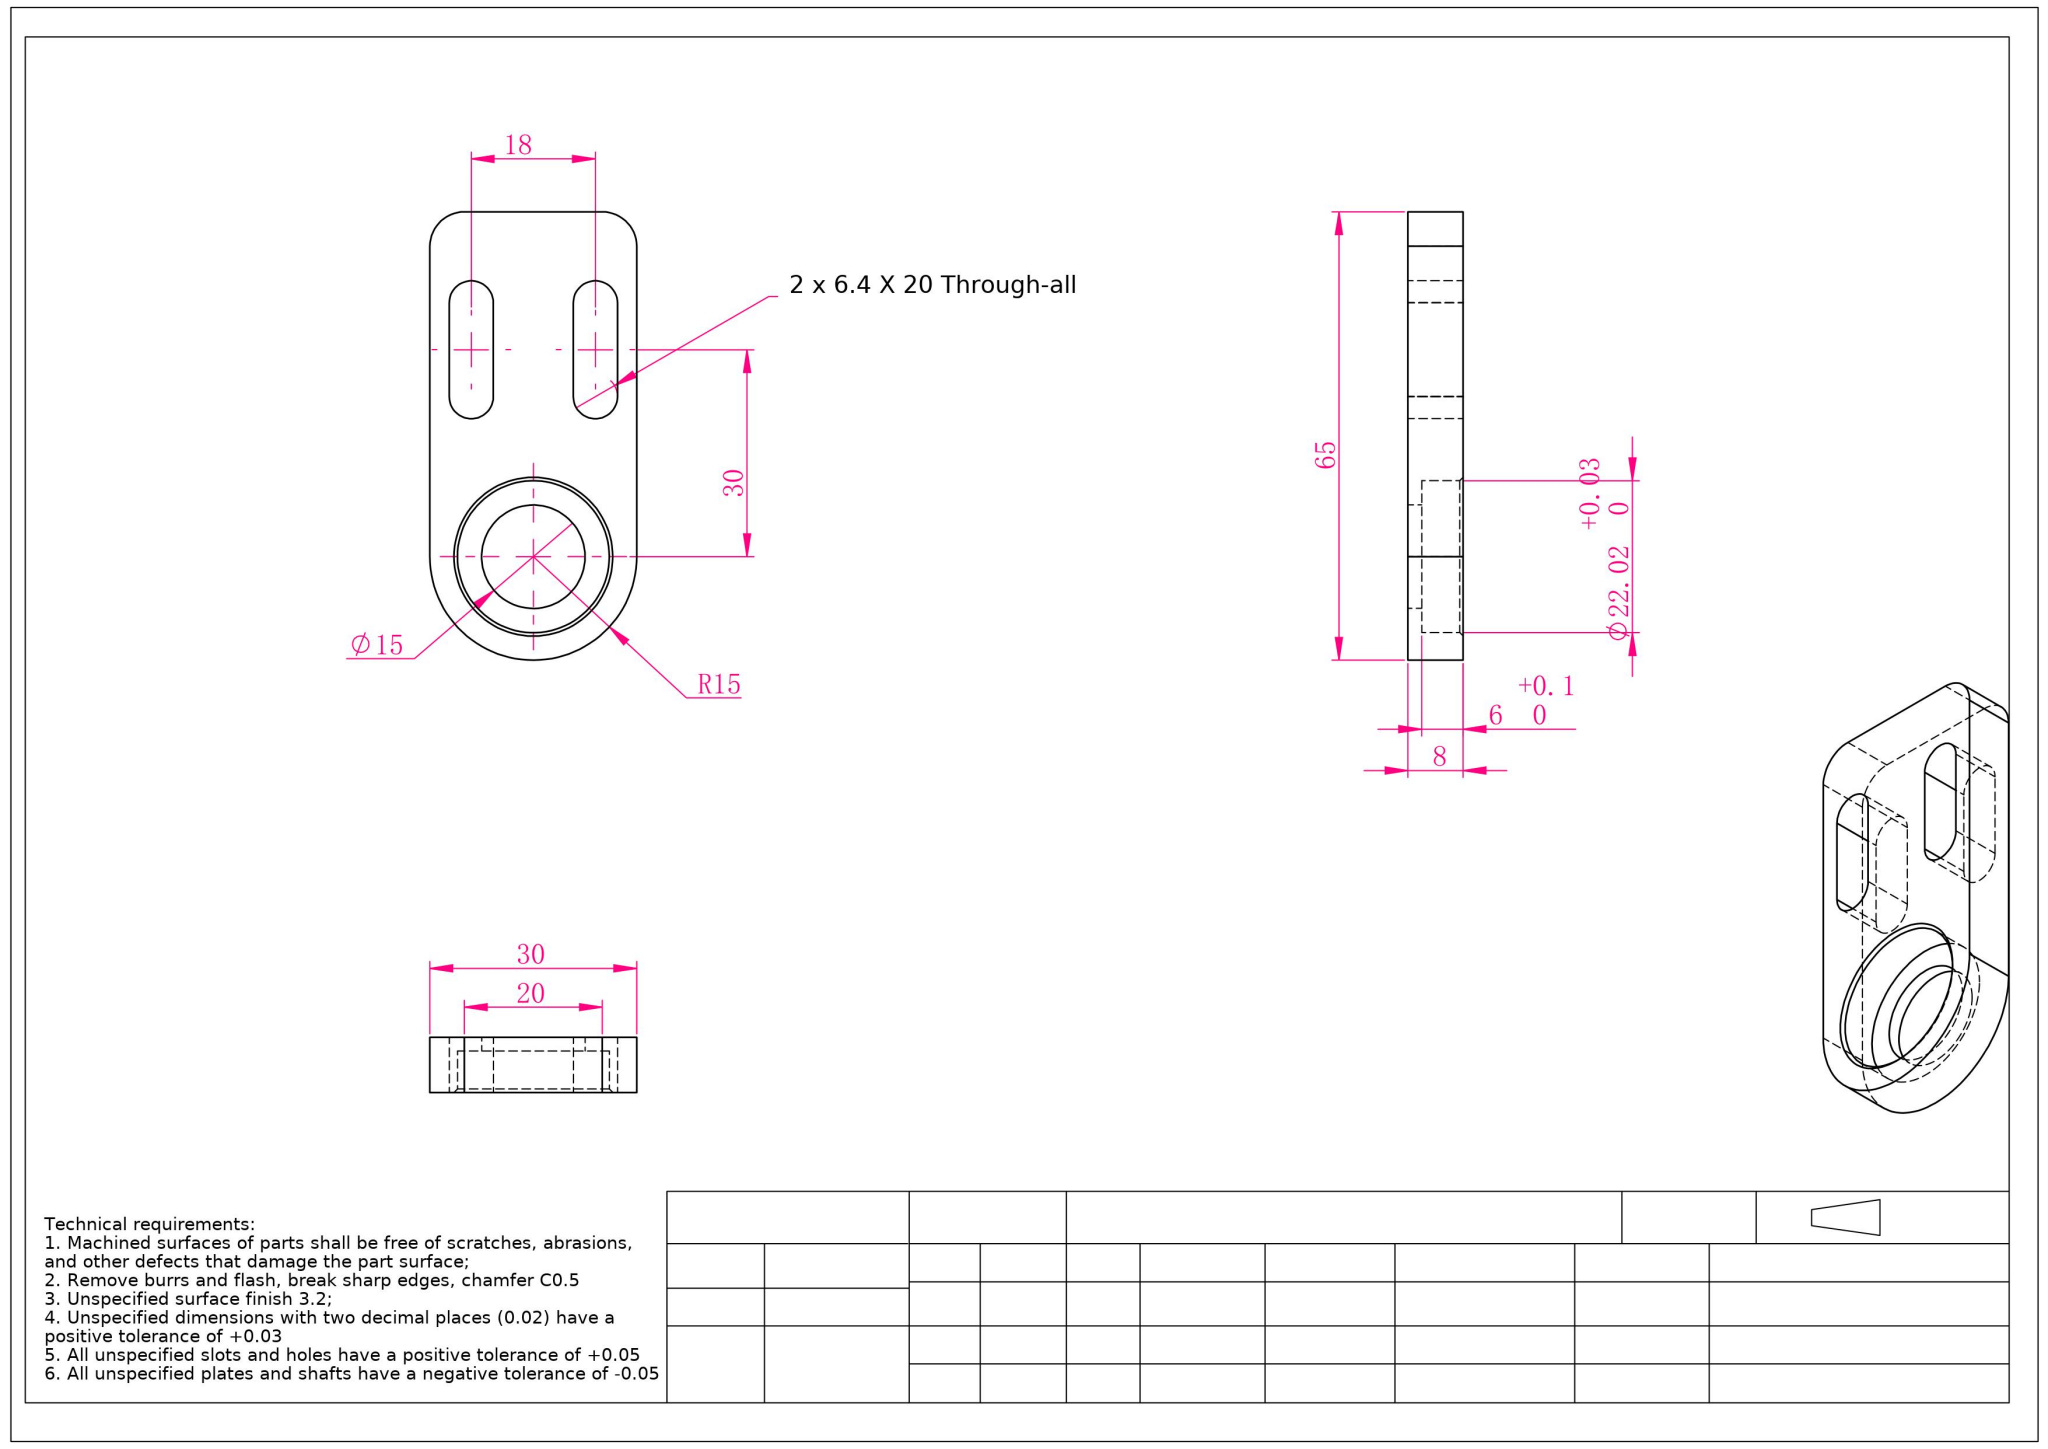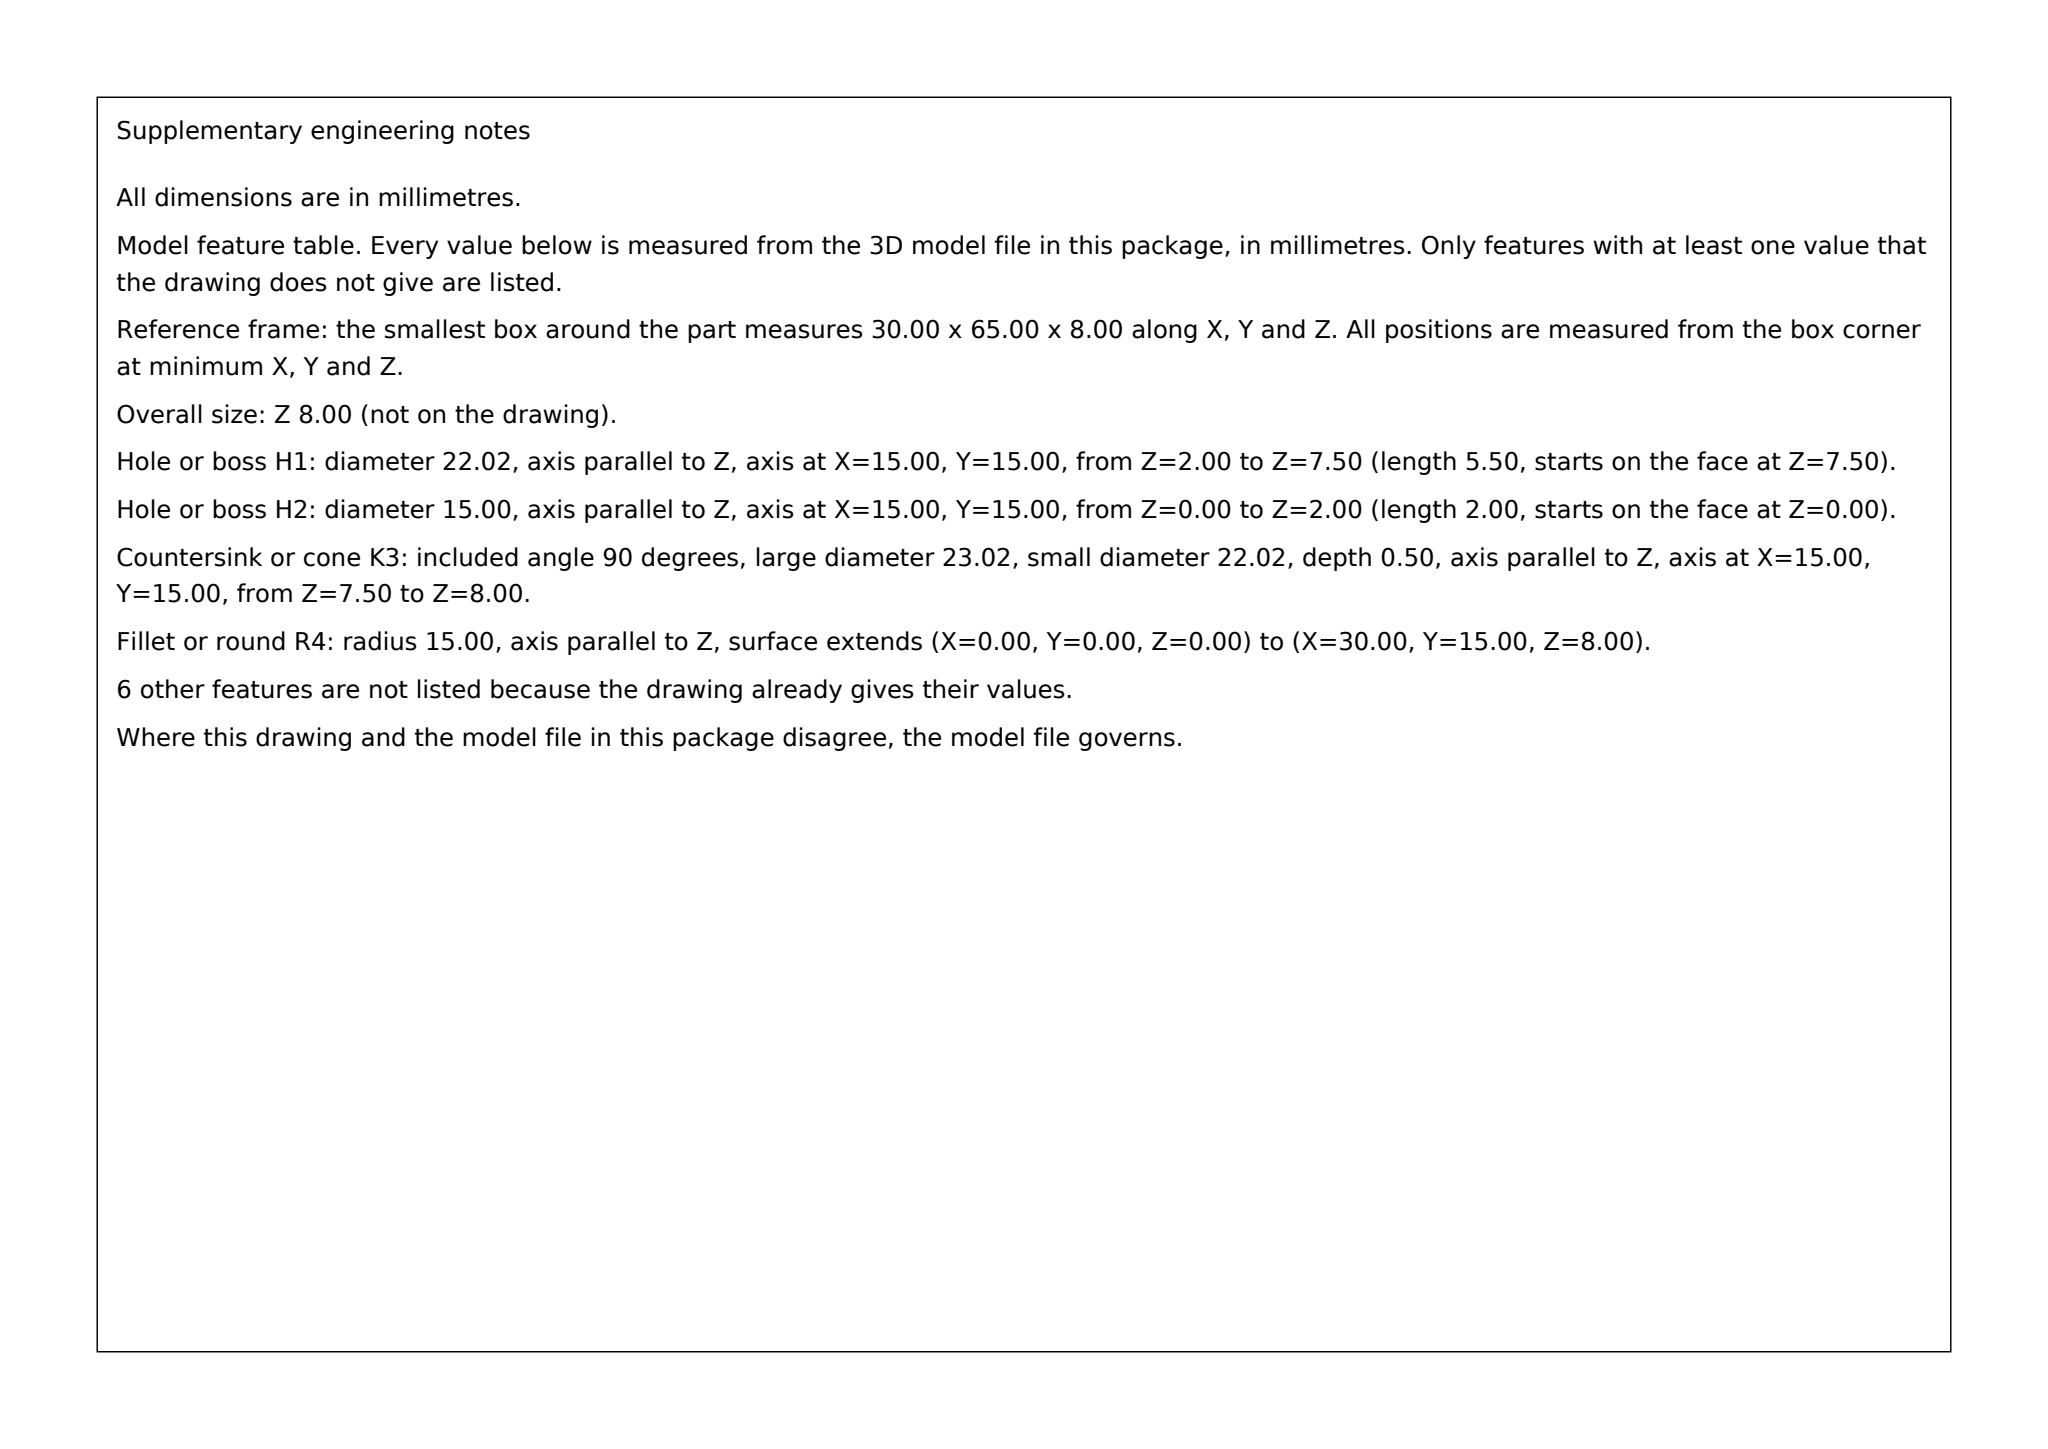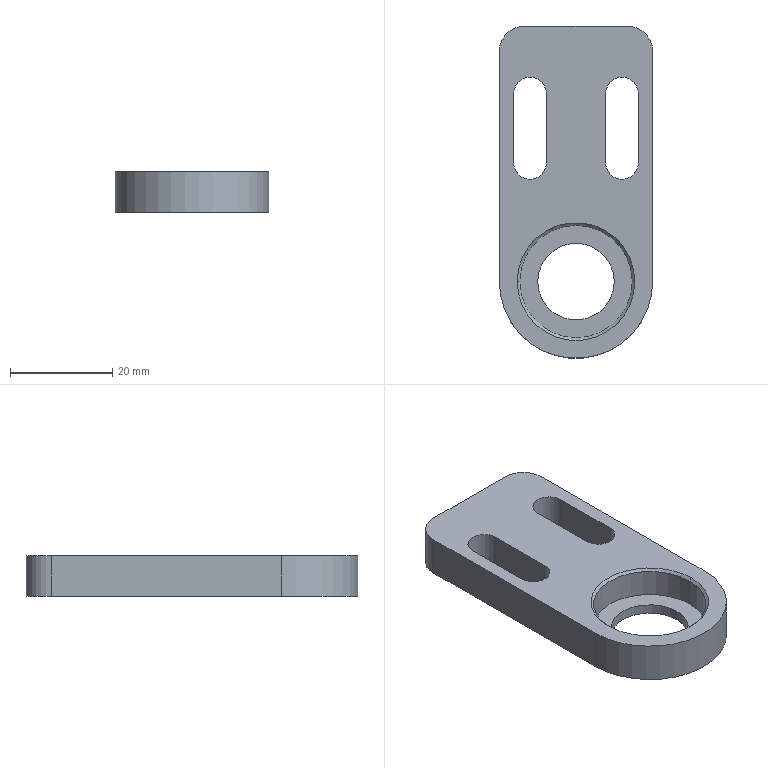Part | SolidWorks | mm | 1 solid | 23 faces | box 30 x 65 x 8 mm | volume 10187 mm3 | cylinder 11 | plane 10 | cone 2 | commonest cylinder face diameters 6.4 x4 22.02 x2 15 x2 10 x2 30 x1
STEP:
#1=CARTESIAN_POINT('',(-11.01,0.,3.5));
#2=VERTEX_POINT('',#1);
#3=CARTESIAN_POINT('',(11.01,0.,3.5));
#4=VERTEX_POINT('',#3);
#5=CARTESIAN_POINT('',(0.,0.,3.5));
#6=DIRECTION('',(0.,0.,1.));
#7=DIRECTION('',(1.,0.,0.));
#8=AXIS2_PLACEMENT_3D('',#5,#6,#7);
#9=CIRCLE('',#8,11.01);
#10=EDGE_CURVE('',#2,#4,#9,.T.);
#11=ORIENTED_EDGE('',*,*,#10,.F.);
#12=CARTESIAN_POINT('',(-11.51,0.,4.));
#13=VERTEX_POINT('',#12);
#14=CARTESIAN_POINT('',(-11.01,0.,3.5));
#15=DIRECTION('',(-0.7071,0.,0.7071));
#16=VECTOR('',#15,1000.);
#17=LINE('',#14,#16);
#18=EDGE_CURVE('',#2,#13,#17,.T.);
#19=ORIENTED_EDGE('',*,*,#18,.T.);
#20=CARTESIAN_POINT('',(11.51,0.,4.));
#21=VERTEX_POINT('',#20);
#22=CARTESIAN_POINT('',(0.,0.,4.));
#23=DIRECTION('',(0.,0.,-1.));
#24=DIRECTION('',(1.,0.,0.));
#25=AXIS2_PLACEMENT_3D('',#22,#23,#24);
#26=CIRCLE('',#25,11.51);
#27=EDGE_CURVE('',#21,#13,#26,.T.);
#28=ORIENTED_EDGE('',*,*,#27,.F.);
#29=CARTESIAN_POINT('',(11.01,0.,3.5));
#30=DIRECTION('',(0.7071,0.,0.7071));
#31=VECTOR('',#30,1000.);
#32=LINE('',#29,#31);
#33=EDGE_CURVE('',#4,#21,#32,.T.);
#34=ORIENTED_EDGE('',*,*,#33,.F.);
#35=EDGE_LOOP('',(#11,#19,#28,#34));
#36=FACE_OUTER_BOUND('',#35,.T.);
#37=CARTESIAN_POINT('',(0.,0.,3.5));
#38=DIRECTION('',(0.,0.,1.));
#39=DIRECTION('',(1.,0.,0.));
#40=AXIS2_PLACEMENT_3D('',#37,#38,#39);
#41=CONICAL_SURFACE('',#40,11.01,0.7854);
#42=ADVANCED_FACE('',(#36),#41,.F.);
#43=CARTESIAN_POINT('',(-11.01,0.,-2.));
#44=VERTEX_POINT('',#43);
#45=CARTESIAN_POINT('',(11.01,0.,-2.));
#46=VERTEX_POINT('',#45);
#47=CARTESIAN_POINT('',(0.,0.,-2.));
#48=DIRECTION('',(0.,0.,1.));
#49=DIRECTION('',(1.,0.,0.));
#50=AXIS2_PLACEMENT_3D('',#47,#48,#49);
#51=CIRCLE('',#50,11.01);
#52=EDGE_CURVE('',#44,#46,#51,.T.);
#53=ORIENTED_EDGE('',*,*,#52,.F.);
#54=CARTESIAN_POINT('',(-11.01,0.,-2.));
#55=DIRECTION('',(0.,0.,1.));
#56=VECTOR('',#55,1000.);
#57=LINE('',#54,#56);
#58=EDGE_CURVE('',#44,#2,#57,.T.);
#59=ORIENTED_EDGE('',*,*,#58,.T.);
#60=ORIENTED_EDGE('',*,*,#10,.T.);
#61=CARTESIAN_POINT('',(11.01,0.,-2.));
#62=DIRECTION('',(0.,0.,1.));
#63=VECTOR('',#62,1000.);
#64=LINE('',#61,#63);
#65=EDGE_CURVE('',#46,#4,#64,.T.);
#66=ORIENTED_EDGE('',*,*,#65,.F.);
#67=EDGE_LOOP('',(#53,#59,#60,#66));
#68=FACE_OUTER_BOUND('',#67,.T.);
#69=CARTESIAN_POINT('',(0.,0.,-2.));
#70=DIRECTION('',(0.,0.,1.));
#71=DIRECTION('',(1.,0.,0.));
#72=AXIS2_PLACEMENT_3D('',#69,#70,#71);
#73=CYLINDRICAL_SURFACE('',#72,11.01);
#74=ADVANCED_FACE('',(#68),#73,.F.);
#75=CARTESIAN_POINT('',(-7.5,0.,-2.));
#76=VERTEX_POINT('',#75);
#77=CARTESIAN_POINT('',(7.5,0.,-2.));
#78=VERTEX_POINT('',#77);
#79=CARTESIAN_POINT('',(0.,0.,-2.));
#80=DIRECTION('',(0.,0.,1.));
#81=DIRECTION('',(1.,0.,0.));
#82=AXIS2_PLACEMENT_3D('',#79,#80,#81);
#83=CIRCLE('',#82,7.5);
#84=EDGE_CURVE('',#76,#78,#83,.T.);
#85=ORIENTED_EDGE('',*,*,#84,.T.);
#86=CARTESIAN_POINT('',(7.5,0.,-4.));
#87=VERTEX_POINT('',#86);
#88=CARTESIAN_POINT('',(7.5,0.,4.));
#89=DIRECTION('',(0.,0.,-1.));
#90=VECTOR('',#89,1000.);
#91=LINE('',#88,#90);
#92=EDGE_CURVE('',#78,#87,#91,.T.);
#93=ORIENTED_EDGE('',*,*,#92,.T.);
#94=CARTESIAN_POINT('',(-7.5,0.,-4.));
#95=VERTEX_POINT('',#94);
#96=CARTESIAN_POINT('',(0.,0.,-4.));
#97=DIRECTION('',(0.,0.,1.));
#98=DIRECTION('',(1.,0.,0.));
#99=AXIS2_PLACEMENT_3D('',#96,#97,#98);
#100=CIRCLE('',#99,7.5);
#101=EDGE_CURVE('',#95,#87,#100,.T.);
#102=ORIENTED_EDGE('',*,*,#101,.F.);
#103=CARTESIAN_POINT('',(-7.5,0.,4.));
#104=DIRECTION('',(0.,0.,-1.));
#105=VECTOR('',#104,1000.);
#106=LINE('',#103,#105);
#107=EDGE_CURVE('',#76,#95,#106,.T.);
#108=ORIENTED_EDGE('',*,*,#107,.F.);
#109=EDGE_LOOP('',(#85,#93,#102,#108));
#110=FACE_OUTER_BOUND('',#109,.T.);
#111=CARTESIAN_POINT('',(0.,0.,4.));
#112=DIRECTION('',(0.,0.,-1.));
#113=DIRECTION('',(-1.,0.,0.));
#114=AXIS2_PLACEMENT_3D('',#111,#112,#113);
#115=CYLINDRICAL_SURFACE('',#114,7.5);
#116=ADVANCED_FACE('',(#110),#115,.F.);
#117=CARTESIAN_POINT('',(12.2,23.2,-4.));
#118=VERTEX_POINT('',#117);
#119=CARTESIAN_POINT('',(5.8,23.2,-4.));
#120=VERTEX_POINT('',#119);
#121=CARTESIAN_POINT('',(9.,23.2,-4.));
#122=DIRECTION('',(0.,0.,-1.));
#123=DIRECTION('',(-1.,0.,0.));
#124=AXIS2_PLACEMENT_3D('',#121,#122,#123);
#125=CIRCLE('',#124,3.2);
#126=EDGE_CURVE('',#118,#120,#125,.T.);
#127=ORIENTED_EDGE('',*,*,#126,.F.);
#128=CARTESIAN_POINT('',(12.2,36.8,-4.));
#129=VERTEX_POINT('',#128);
#130=CARTESIAN_POINT('',(12.2,23.2,-4.));
#131=DIRECTION('',(0.,1.,0.));
#132=VECTOR('',#131,1000.);
#133=LINE('',#130,#132);
#134=EDGE_CURVE('',#118,#129,#133,.T.);
#135=ORIENTED_EDGE('',*,*,#134,.T.);
#136=CARTESIAN_POINT('',(5.8,36.8,-4.));
#137=VERTEX_POINT('',#136);
#138=CARTESIAN_POINT('',(9.,36.8,-4.));
#139=DIRECTION('',(0.,0.,-1.));
#140=DIRECTION('',(-1.,0.,0.));
#141=AXIS2_PLACEMENT_3D('',#138,#139,#140);
#142=CIRCLE('',#141,3.2);
#143=EDGE_CURVE('',#137,#129,#142,.T.);
#144=ORIENTED_EDGE('',*,*,#143,.F.);
#145=CARTESIAN_POINT('',(5.8,23.2,-4.));
#146=DIRECTION('',(0.,1.,0.));
#147=VECTOR('',#146,1000.);
#148=LINE('',#145,#147);
#149=EDGE_CURVE('',#120,#137,#148,.T.);
#150=ORIENTED_EDGE('',*,*,#149,.F.);
#151=EDGE_LOOP('',(#127,#135,#144,#150));
#152=FACE_BOUND('',#151,.T.);
#153=ORIENTED_EDGE('',*,*,#101,.T.);
#154=CARTESIAN_POINT('',(0.,0.,-4.));
#155=DIRECTION('',(0.,0.,1.));
#156=DIRECTION('',(1.,0.,0.));
#157=AXIS2_PLACEMENT_3D('',#154,#155,#156);
#158=CIRCLE('',#157,7.5);
#159=EDGE_CURVE('',#87,#95,#158,.T.);
#160=ORIENTED_EDGE('',*,*,#159,.T.);
#161=EDGE_LOOP('',(#153,#160));
#162=FACE_BOUND('',#161,.T.);
#163=CARTESIAN_POINT('',(10.,50.,-4.));
#164=VERTEX_POINT('',#163);
#165=CARTESIAN_POINT('',(-10.,50.,-4.));
#166=VERTEX_POINT('',#165);
#167=CARTESIAN_POINT('',(-15.,50.,-4.));
#168=DIRECTION('',(-1.,0.,0.));
#169=VECTOR('',#168,1000.);
#170=LINE('',#167,#169);
#171=EDGE_CURVE('',#164,#166,#170,.T.);
#172=ORIENTED_EDGE('',*,*,#171,.F.);
#173=CARTESIAN_POINT('',(15.,45.,-4.));
#174=VERTEX_POINT('',#173);
#175=CARTESIAN_POINT('',(10.,45.,-4.));
#176=DIRECTION('',(0.,0.,-1.));
#177=DIRECTION('',(1.,0.,0.));
#178=AXIS2_PLACEMENT_3D('',#175,#176,#177);
#179=CIRCLE('',#178,5.);
#180=EDGE_CURVE('',#164,#174,#179,.T.);
#181=ORIENTED_EDGE('',*,*,#180,.T.);
#182=CARTESIAN_POINT('',(15.,-0.,-4.));
#183=VERTEX_POINT('',#182);
#184=CARTESIAN_POINT('',(15.,50.,-4.));
#185=DIRECTION('',(0.,1.,0.));
#186=VECTOR('',#185,1000.);
#187=LINE('',#184,#186);
#188=EDGE_CURVE('',#183,#174,#187,.T.);
#189=ORIENTED_EDGE('',*,*,#188,.F.);
#190=CARTESIAN_POINT('',(-15.,-0.,-4.));
#191=VERTEX_POINT('',#190);
#192=CARTESIAN_POINT('',(0.,0.,-4.));
#193=DIRECTION('',(0.,0.,1.));
#194=DIRECTION('',(1.,0.,0.));
#195=AXIS2_PLACEMENT_3D('',#192,#193,#194);
#196=CIRCLE('',#195,15.);
#197=EDGE_CURVE('',#191,#183,#196,.T.);
#198=ORIENTED_EDGE('',*,*,#197,.F.);
#199=CARTESIAN_POINT('',(-15.,45.,-4.));
#200=VERTEX_POINT('',#199);
#201=CARTESIAN_POINT('',(-15.,50.,-4.));
#202=DIRECTION('',(0.,-1.,0.));
#203=VECTOR('',#202,1000.);
#204=LINE('',#201,#203);
#205=EDGE_CURVE('',#200,#191,#204,.T.);
#206=ORIENTED_EDGE('',*,*,#205,.F.);
#207=CARTESIAN_POINT('',(-10.,45.,-4.));
#208=DIRECTION('',(0.,0.,-1.));
#209=DIRECTION('',(1.,0.,0.));
#210=AXIS2_PLACEMENT_3D('',#207,#208,#209);
#211=CIRCLE('',#210,5.);
#212=EDGE_CURVE('',#200,#166,#211,.T.);
#213=ORIENTED_EDGE('',*,*,#212,.T.);
#214=EDGE_LOOP('',(#172,#181,#189,#198,#206,#213));
#215=FACE_OUTER_BOUND('',#214,.T.);
#216=CARTESIAN_POINT('',(-12.2,36.8,-4.));
#217=VERTEX_POINT('',#216);
#218=CARTESIAN_POINT('',(-5.8,36.8,-4.));
#219=VERTEX_POINT('',#218);
#220=CARTESIAN_POINT('',(-9.,36.8,-4.));
#221=DIRECTION('',(0.,0.,-1.));
#222=DIRECTION('',(-1.,0.,0.));
#223=AXIS2_PLACEMENT_3D('',#220,#221,#222);
#224=CIRCLE('',#223,3.2);
#225=EDGE_CURVE('',#217,#219,#224,.T.);
#226=ORIENTED_EDGE('',*,*,#225,.F.);
#227=CARTESIAN_POINT('',(-12.2,23.2,-4.));
#228=VERTEX_POINT('',#227);
#229=CARTESIAN_POINT('',(-12.2,23.2,-4.));
#230=DIRECTION('',(0.,1.,0.));
#231=VECTOR('',#230,1000.);
#232=LINE('',#229,#231);
#233=EDGE_CURVE('',#228,#217,#232,.T.);
#234=ORIENTED_EDGE('',*,*,#233,.F.);
#235=CARTESIAN_POINT('',(-5.8,23.2,-4.));
#236=VERTEX_POINT('',#235);
#237=CARTESIAN_POINT('',(-9.,23.2,-4.));
#238=DIRECTION('',(0.,0.,-1.));
#239=DIRECTION('',(-1.,0.,0.));
#240=AXIS2_PLACEMENT_3D('',#237,#238,#239);
#241=CIRCLE('',#240,3.2);
#242=EDGE_CURVE('',#236,#228,#241,.T.);
#243=ORIENTED_EDGE('',*,*,#242,.F.);
#244=CARTESIAN_POINT('',(-5.8,23.2,-4.));
#245=DIRECTION('',(0.,1.,0.));
#246=VECTOR('',#245,1000.);
#247=LINE('',#244,#246);
#248=EDGE_CURVE('',#236,#219,#247,.T.);
#249=ORIENTED_EDGE('',*,*,#248,.T.);
#250=EDGE_LOOP('',(#226,#234,#243,#249));
#251=FACE_BOUND('',#250,.T.);
#252=CARTESIAN_POINT('',(0.,0.,-4.));
#253=DIRECTION('',(0.,0.,1.));
#254=DIRECTION('',(1.,0.,0.));
#255=AXIS2_PLACEMENT_3D('',#252,#253,#254);
#256=PLANE('',#255);
#257=ADVANCED_FACE('',(#152,#162,#215,#251),#256,.F.);
#258=ORIENTED_EDGE('',*,*,#92,.F.);
#259=CARTESIAN_POINT('',(0.,0.,-2.));
#260=DIRECTION('',(0.,0.,1.));
#261=DIRECTION('',(1.,0.,0.));
#262=AXIS2_PLACEMENT_3D('',#259,#260,#261);
#263=CIRCLE('',#262,7.5);
#264=EDGE_CURVE('',#78,#76,#263,.T.);
#265=ORIENTED_EDGE('',*,*,#264,.T.);
#266=ORIENTED_EDGE('',*,*,#107,.T.);
#267=ORIENTED_EDGE('',*,*,#159,.F.);
#268=EDGE_LOOP('',(#258,#265,#266,#267));
#269=FACE_OUTER_BOUND('',#268,.T.);
#270=CARTESIAN_POINT('',(0.,0.,4.));
#271=DIRECTION('',(0.,0.,-1.));
#272=DIRECTION('',(-1.,0.,0.));
#273=AXIS2_PLACEMENT_3D('',#270,#271,#272);
#274=CYLINDRICAL_SURFACE('',#273,7.5);
#275=ADVANCED_FACE('',(#269),#274,.F.);
#276=CARTESIAN_POINT('',(12.2,23.2,4.));
#277=VERTEX_POINT('',#276);
#278=CARTESIAN_POINT('',(12.2,36.8,4.));
#279=VERTEX_POINT('',#278);
#280=CARTESIAN_POINT('',(12.2,23.2,4.));
#281=DIRECTION('',(0.,1.,0.));
#282=VECTOR('',#281,1000.);
#283=LINE('',#280,#282);
#284=EDGE_CURVE('',#277,#279,#283,.T.);
#285=ORIENTED_EDGE('',*,*,#284,.F.);
#286=CARTESIAN_POINT('',(5.8,23.2,4.));
#287=VERTEX_POINT('',#286);
#288=CARTESIAN_POINT('',(9.,23.2,4.));
#289=DIRECTION('',(0.,0.,-1.));
#290=DIRECTION('',(-1.,0.,0.));
#291=AXIS2_PLACEMENT_3D('',#288,#289,#290);
#292=CIRCLE('',#291,3.2);
#293=EDGE_CURVE('',#277,#287,#292,.T.);
#294=ORIENTED_EDGE('',*,*,#293,.T.);
#295=CARTESIAN_POINT('',(5.8,36.8,4.));
#296=VERTEX_POINT('',#295);
#297=CARTESIAN_POINT('',(5.8,23.2,4.));
#298=DIRECTION('',(0.,1.,0.));
#299=VECTOR('',#298,1000.);
#300=LINE('',#297,#299);
#301=EDGE_CURVE('',#287,#296,#300,.T.);
#302=ORIENTED_EDGE('',*,*,#301,.T.);
#303=CARTESIAN_POINT('',(9.,36.8,4.));
#304=DIRECTION('',(0.,0.,-1.));
#305=DIRECTION('',(-1.,0.,0.));
#306=AXIS2_PLACEMENT_3D('',#303,#304,#305);
#307=CIRCLE('',#306,3.2);
#308=EDGE_CURVE('',#296,#279,#307,.T.);
#309=ORIENTED_EDGE('',*,*,#308,.T.);
#310=EDGE_LOOP('',(#285,#294,#302,#309));
#311=FACE_BOUND('',#310,.T.);
#312=CARTESIAN_POINT('',(-12.2,36.8,4.));
#313=VERTEX_POINT('',#312);
#314=CARTESIAN_POINT('',(-5.8,36.8,4.));
#315=VERTEX_POINT('',#314);
#316=CARTESIAN_POINT('',(-9.,36.8,4.));
#317=DIRECTION('',(0.,0.,-1.));
#318=DIRECTION('',(-1.,0.,0.));
#319=AXIS2_PLACEMENT_3D('',#316,#317,#318);
#320=CIRCLE('',#319,3.2);
#321=EDGE_CURVE('',#313,#315,#320,.T.);
#322=ORIENTED_EDGE('',*,*,#321,.T.);
#323=CARTESIAN_POINT('',(-5.8,23.2,4.));
#324=VERTEX_POINT('',#323);
#325=CARTESIAN_POINT('',(-5.8,23.2,4.));
#326=DIRECTION('',(0.,1.,0.));
#327=VECTOR('',#326,1000.);
#328=LINE('',#325,#327);
#329=EDGE_CURVE('',#324,#315,#328,.T.);
#330=ORIENTED_EDGE('',*,*,#329,.F.);
#331=CARTESIAN_POINT('',(-12.2,23.2,4.));
#332=VERTEX_POINT('',#331);
#333=CARTESIAN_POINT('',(-9.,23.2,4.));
#334=DIRECTION('',(0.,0.,-1.));
#335=DIRECTION('',(-1.,0.,0.));
#336=AXIS2_PLACEMENT_3D('',#333,#334,#335);
#337=CIRCLE('',#336,3.2);
#338=EDGE_CURVE('',#324,#332,#337,.T.);
#339=ORIENTED_EDGE('',*,*,#338,.T.);
#340=CARTESIAN_POINT('',(-12.2,23.2,4.));
#341=DIRECTION('',(0.,1.,0.));
#342=VECTOR('',#341,1000.);
#343=LINE('',#340,#342);
#344=EDGE_CURVE('',#332,#313,#343,.T.);
#345=ORIENTED_EDGE('',*,*,#344,.T.);
#346=EDGE_LOOP('',(#322,#330,#339,#345));
#347=FACE_BOUND('',#346,.T.);
#348=ORIENTED_EDGE('',*,*,#27,.T.);
#349=CARTESIAN_POINT('',(0.,0.,4.));
#350=DIRECTION('',(0.,0.,-1.));
#351=DIRECTION('',(1.,0.,0.));
#352=AXIS2_PLACEMENT_3D('',#349,#350,#351);
#353=CIRCLE('',#352,11.51);
#354=EDGE_CURVE('',#13,#21,#353,.T.);
#355=ORIENTED_EDGE('',*,*,#354,.T.);
#356=EDGE_LOOP('',(#348,#355));
#357=FACE_BOUND('',#356,.T.);
#358=CARTESIAN_POINT('',(15.,-0.,4.));
#359=VERTEX_POINT('',#358);
#360=CARTESIAN_POINT('',(15.,45.,4.));
#361=VERTEX_POINT('',#360);
#362=CARTESIAN_POINT('',(15.,50.,4.));
#363=DIRECTION('',(0.,1.,0.));
#364=VECTOR('',#363,1000.);
#365=LINE('',#362,#364);
#366=EDGE_CURVE('',#359,#361,#365,.T.);
#367=ORIENTED_EDGE('',*,*,#366,.T.);
#368=CARTESIAN_POINT('',(10.,50.,4.));
#369=VERTEX_POINT('',#368);
#370=CARTESIAN_POINT('',(10.,45.,4.));
#371=DIRECTION('',(0.,0.,1.));
#372=DIRECTION('',(1.,0.,0.));
#373=AXIS2_PLACEMENT_3D('',#370,#371,#372);
#374=CIRCLE('',#373,5.);
#375=EDGE_CURVE('',#361,#369,#374,.T.);
#376=ORIENTED_EDGE('',*,*,#375,.T.);
#377=CARTESIAN_POINT('',(-10.,50.,4.));
#378=VERTEX_POINT('',#377);
#379=CARTESIAN_POINT('',(-15.,50.,4.));
#380=DIRECTION('',(-1.,0.,0.));
#381=VECTOR('',#380,1000.);
#382=LINE('',#379,#381);
#383=EDGE_CURVE('',#369,#378,#382,.T.);
#384=ORIENTED_EDGE('',*,*,#383,.T.);
#385=CARTESIAN_POINT('',(-15.,45.,4.));
#386=VERTEX_POINT('',#385);
#387=CARTESIAN_POINT('',(-10.,45.,4.));
#388=DIRECTION('',(0.,0.,1.));
#389=DIRECTION('',(1.,0.,0.));
#390=AXIS2_PLACEMENT_3D('',#387,#388,#389);
#391=CIRCLE('',#390,5.);
#392=EDGE_CURVE('',#378,#386,#391,.T.);
#393=ORIENTED_EDGE('',*,*,#392,.T.);
#394=CARTESIAN_POINT('',(-15.,-0.,4.));
#395=VERTEX_POINT('',#394);
#396=CARTESIAN_POINT('',(-15.,50.,4.));
#397=DIRECTION('',(0.,-1.,0.));
#398=VECTOR('',#397,1000.);
#399=LINE('',#396,#398);
#400=EDGE_CURVE('',#386,#395,#399,.T.);
#401=ORIENTED_EDGE('',*,*,#400,.T.);
#402=CARTESIAN_POINT('',(0.,0.,4.));
#403=DIRECTION('',(0.,0.,1.));
#404=DIRECTION('',(1.,0.,0.));
#405=AXIS2_PLACEMENT_3D('',#402,#403,#404);
#406=CIRCLE('',#405,15.);
#407=EDGE_CURVE('',#395,#359,#406,.T.);
#408=ORIENTED_EDGE('',*,*,#407,.T.);
#409=EDGE_LOOP('',(#367,#376,#384,#393,#401,#408));
#410=FACE_OUTER_BOUND('',#409,.T.);
#411=CARTESIAN_POINT('',(0.,0.,4.));
#412=DIRECTION('',(0.,0.,1.));
#413=DIRECTION('',(1.,0.,0.));
#414=AXIS2_PLACEMENT_3D('',#411,#412,#413);
#415=PLANE('',#414);
#416=ADVANCED_FACE('',(#311,#347,#357,#410),#415,.T.);
#417=ORIENTED_EDGE('',*,*,#197,.T.);
#418=CARTESIAN_POINT('',(15.,-0.,4.));
#419=DIRECTION('',(0.,0.,-1.));
#420=VECTOR('',#419,1000.);
#421=LINE('',#418,#420);
#422=EDGE_CURVE('',#359,#183,#421,.T.);
#423=ORIENTED_EDGE('',*,*,#422,.F.);
#424=ORIENTED_EDGE('',*,*,#407,.F.);
#425=CARTESIAN_POINT('',(-15.,-0.,4.));
#426=DIRECTION('',(0.,0.,-1.));
#427=VECTOR('',#426,1000.);
#428=LINE('',#425,#427);
#429=EDGE_CURVE('',#395,#191,#428,.T.);
#430=ORIENTED_EDGE('',*,*,#429,.T.);
#431=EDGE_LOOP('',(#417,#423,#424,#430));
#432=FACE_OUTER_BOUND('',#431,.T.);
#433=CARTESIAN_POINT('',(0.,0.,4.));
#434=DIRECTION('',(0.,0.,-1.));
#435=DIRECTION('',(-1.,0.,0.));
#436=AXIS2_PLACEMENT_3D('',#433,#434,#435);
#437=CYLINDRICAL_SURFACE('',#436,15.);
#438=ADVANCED_FACE('',(#432),#437,.T.);
#439=ORIENTED_EDGE('',*,*,#188,.T.);
#440=CARTESIAN_POINT('',(15.,45.,4.));
#441=DIRECTION('',(0.,0.,1.));
#442=VECTOR('',#441,1000.);
#443=LINE('',#440,#442);
#444=EDGE_CURVE('',#174,#361,#443,.T.);
#445=ORIENTED_EDGE('',*,*,#444,.T.);
#446=ORIENTED_EDGE('',*,*,#366,.F.);
#447=ORIENTED_EDGE('',*,*,#422,.T.);
#448=EDGE_LOOP('',(#439,#445,#446,#447));
#449=FACE_OUTER_BOUND('',#448,.T.);
#450=CARTESIAN_POINT('',(15.,50.,4.));
#451=DIRECTION('',(-1.,0.,0.));
#452=DIRECTION('',(-0.,-1.,0.));
#453=AXIS2_PLACEMENT_3D('',#450,#451,#452);
#454=PLANE('',#453);
#455=ADVANCED_FACE('',(#449),#454,.F.);
#456=ORIENTED_EDGE('',*,*,#383,.F.);
#457=CARTESIAN_POINT('',(10.,50.,4.));
#458=DIRECTION('',(0.,0.,-1.));
#459=VECTOR('',#458,1000.);
#460=LINE('',#457,#459);
#461=EDGE_CURVE('',#369,#164,#460,.T.);
#462=ORIENTED_EDGE('',*,*,#461,.T.);
#463=ORIENTED_EDGE('',*,*,#171,.T.);
#464=CARTESIAN_POINT('',(-10.,50.,4.));
#465=DIRECTION('',(0.,0.,1.));
#466=VECTOR('',#465,1000.);
#467=LINE('',#464,#466);
#468=EDGE_CURVE('',#166,#378,#467,.T.);
#469=ORIENTED_EDGE('',*,*,#468,.T.);
#470=EDGE_LOOP('',(#456,#462,#463,#469));
#471=FACE_OUTER_BOUND('',#470,.T.);
#472=CARTESIAN_POINT('',(-15.,50.,4.));
#473=DIRECTION('',(0.,-1.,0.));
#474=DIRECTION('',(0.,0.,-1.));
#475=AXIS2_PLACEMENT_3D('',#472,#473,#474);
#476=PLANE('',#475);
#477=ADVANCED_FACE('',(#471),#476,.F.);
#478=ORIENTED_EDGE('',*,*,#400,.F.);
#479=CARTESIAN_POINT('',(-15.,45.,4.));
#480=DIRECTION('',(0.,0.,-1.));
#481=VECTOR('',#480,1000.);
#482=LINE('',#479,#481);
#483=EDGE_CURVE('',#386,#200,#482,.T.);
#484=ORIENTED_EDGE('',*,*,#483,.T.);
#485=ORIENTED_EDGE('',*,*,#205,.T.);
#486=ORIENTED_EDGE('',*,*,#429,.F.);
#487=EDGE_LOOP('',(#478,#484,#485,#486));
#488=FACE_OUTER_BOUND('',#487,.T.);
#489=CARTESIAN_POINT('',(-15.,50.,4.));
#490=DIRECTION('',(1.,0.,0.));
#491=DIRECTION('',(-0.,1.,0.));
#492=AXIS2_PLACEMENT_3D('',#489,#490,#491);
#493=PLANE('',#492);
#494=ADVANCED_FACE('',(#488),#493,.F.);
#495=ORIENTED_EDGE('',*,*,#58,.F.);
#496=CARTESIAN_POINT('',(0.,0.,-2.));
#497=DIRECTION('',(0.,0.,1.));
#498=DIRECTION('',(1.,0.,0.));
#499=AXIS2_PLACEMENT_3D('',#496,#497,#498);
#500=CIRCLE('',#499,11.01);
#501=EDGE_CURVE('',#46,#44,#500,.T.);
#502=ORIENTED_EDGE('',*,*,#501,.F.);
#503=ORIENTED_EDGE('',*,*,#65,.T.);
#504=CARTESIAN_POINT('',(0.,0.,3.5));
#505=DIRECTION('',(0.,0.,1.));
#506=DIRECTION('',(1.,0.,0.));
#507=AXIS2_PLACEMENT_3D('',#504,#505,#506);
#508=CIRCLE('',#507,11.01);
#509=EDGE_CURVE('',#4,#2,#508,.T.);
#510=ORIENTED_EDGE('',*,*,#509,.T.);
#511=EDGE_LOOP('',(#495,#502,#503,#510));
#512=FACE_OUTER_BOUND('',#511,.T.);
#513=CARTESIAN_POINT('',(0.,0.,-2.));
#514=DIRECTION('',(0.,0.,1.));
#515=DIRECTION('',(1.,0.,0.));
#516=AXIS2_PLACEMENT_3D('',#513,#514,#515);
#517=CYLINDRICAL_SURFACE('',#516,11.01);
#518=ADVANCED_FACE('',(#512),#517,.F.);
#519=ORIENTED_EDGE('',*,*,#84,.F.);
#520=ORIENTED_EDGE('',*,*,#264,.F.);
#521=EDGE_LOOP('',(#519,#520));
#522=FACE_BOUND('',#521,.T.);
#523=ORIENTED_EDGE('',*,*,#501,.T.);
#524=ORIENTED_EDGE('',*,*,#52,.T.);
#525=EDGE_LOOP('',(#523,#524));
#526=FACE_OUTER_BOUND('',#525,.T.);
#527=CARTESIAN_POINT('',(0.,0.,-2.));
#528=DIRECTION('',(0.,0.,1.));
#529=DIRECTION('',(1.,0.,0.));
#530=AXIS2_PLACEMENT_3D('',#527,#528,#529);
#531=PLANE('',#530);
#532=ADVANCED_FACE('',(#522,#526),#531,.T.);
#533=ORIENTED_EDGE('',*,*,#18,.F.);
#534=ORIENTED_EDGE('',*,*,#509,.F.);
#535=ORIENTED_EDGE('',*,*,#33,.T.);
#536=ORIENTED_EDGE('',*,*,#354,.F.);
#537=EDGE_LOOP('',(#533,#534,#535,#536));
#538=FACE_OUTER_BOUND('',#537,.T.);
#539=CARTESIAN_POINT('',(0.,0.,3.5));
#540=DIRECTION('',(0.,0.,1.));
#541=DIRECTION('',(1.,0.,0.));
#542=AXIS2_PLACEMENT_3D('',#539,#540,#541);
#543=CONICAL_SURFACE('',#542,11.01,0.7854);
#544=ADVANCED_FACE('',(#538),#543,.F.);
#545=ORIENTED_EDGE('',*,*,#225,.T.);
#546=CARTESIAN_POINT('',(-5.8,36.8,4.));
#547=DIRECTION('',(-0.,0.,1.));
#548=VECTOR('',#547,1000.);
#549=LINE('',#546,#548);
#550=EDGE_CURVE('',#219,#315,#549,.T.);
#551=ORIENTED_EDGE('',*,*,#550,.T.);
#552=ORIENTED_EDGE('',*,*,#321,.F.);
#553=CARTESIAN_POINT('',(-12.2,36.8,-4.));
#554=DIRECTION('',(0.,0.,1.));
#555=VECTOR('',#554,1000.);
#556=LINE('',#553,#555);
#557=EDGE_CURVE('',#217,#313,#556,.T.);
#558=ORIENTED_EDGE('',*,*,#557,.F.);
#559=EDGE_LOOP('',(#545,#551,#552,#558));
#560=FACE_OUTER_BOUND('',#559,.T.);
#561=CARTESIAN_POINT('',(-9.,36.8,-4.));
#562=DIRECTION('',(0.,0.,-1.));
#563=DIRECTION('',(-1.,0.,0.));
#564=AXIS2_PLACEMENT_3D('',#561,#562,#563);
#565=CYLINDRICAL_SURFACE('',#564,3.2);
#566=ADVANCED_FACE('',(#560),#565,.F.);
#567=ORIENTED_EDGE('',*,*,#338,.F.);
#568=CARTESIAN_POINT('',(-5.8,23.2,4.));
#569=DIRECTION('',(-0.,0.,1.));
#570=VECTOR('',#569,1000.);
#571=LINE('',#568,#570);
#572=EDGE_CURVE('',#236,#324,#571,.T.);
#573=ORIENTED_EDGE('',*,*,#572,.F.);
#574=ORIENTED_EDGE('',*,*,#242,.T.);
#575=CARTESIAN_POINT('',(-12.2,23.2,-4.));
#576=DIRECTION('',(0.,0.,-1.));
#577=VECTOR('',#576,1000.);
#578=LINE('',#575,#577);
#579=EDGE_CURVE('',#332,#228,#578,.T.);
#580=ORIENTED_EDGE('',*,*,#579,.F.);
#581=EDGE_LOOP('',(#567,#573,#574,#580));
#582=FACE_OUTER_BOUND('',#581,.T.);
#583=CARTESIAN_POINT('',(-9.,23.2,-4.));
#584=DIRECTION('',(0.,0.,-1.));
#585=DIRECTION('',(-1.,0.,0.));
#586=AXIS2_PLACEMENT_3D('',#583,#584,#585);
#587=CYLINDRICAL_SURFACE('',#586,3.2);
#588=ADVANCED_FACE('',(#582),#587,.F.);
#589=ORIENTED_EDGE('',*,*,#550,.F.);
#590=ORIENTED_EDGE('',*,*,#248,.F.);
#591=ORIENTED_EDGE('',*,*,#572,.T.);
#592=ORIENTED_EDGE('',*,*,#329,.T.);
#593=EDGE_LOOP('',(#589,#590,#591,#592));
#594=FACE_OUTER_BOUND('',#593,.T.);
#595=CARTESIAN_POINT('',(-5.8,23.2,4.));
#596=DIRECTION('',(-1.,0.,-0.));
#597=DIRECTION('',(-0.,-1.,0.));
#598=AXIS2_PLACEMENT_3D('',#595,#596,#597);
#599=PLANE('',#598);
#600=ADVANCED_FACE('',(#594),#599,.T.);
#601=ORIENTED_EDGE('',*,*,#557,.T.);
#602=ORIENTED_EDGE('',*,*,#344,.F.);
#603=ORIENTED_EDGE('',*,*,#579,.T.);
#604=ORIENTED_EDGE('',*,*,#233,.T.);
#605=EDGE_LOOP('',(#601,#602,#603,#604));
#606=FACE_OUTER_BOUND('',#605,.T.);
#607=CARTESIAN_POINT('',(-12.2,23.2,-4.));
#608=DIRECTION('',(-1.,0.,0.));
#609=DIRECTION('',(-0.,-1.,0.));
#610=AXIS2_PLACEMENT_3D('',#607,#608,#609);
#611=PLANE('',#610);
#612=ADVANCED_FACE('',(#606),#611,.F.);
#613=ORIENTED_EDGE('',*,*,#143,.T.);
#614=CARTESIAN_POINT('',(12.2,36.8,4.));
#615=DIRECTION('',(-0.,0.,1.));
#616=VECTOR('',#615,1000.);
#617=LINE('',#614,#616);
#618=EDGE_CURVE('',#129,#279,#617,.T.);
#619=ORIENTED_EDGE('',*,*,#618,.T.);
#620=ORIENTED_EDGE('',*,*,#308,.F.);
#621=CARTESIAN_POINT('',(5.8,36.8,-4.));
#622=DIRECTION('',(0.,0.,1.));
#623=VECTOR('',#622,1000.);
#624=LINE('',#621,#623);
#625=EDGE_CURVE('',#137,#296,#624,.T.);
#626=ORIENTED_EDGE('',*,*,#625,.F.);
#627=EDGE_LOOP('',(#613,#619,#620,#626));
#628=FACE_OUTER_BOUND('',#627,.T.);
#629=CARTESIAN_POINT('',(9.,36.8,-4.));
#630=DIRECTION('',(0.,0.,-1.));
#631=DIRECTION('',(-1.,0.,0.));
#632=AXIS2_PLACEMENT_3D('',#629,#630,#631);
#633=CYLINDRICAL_SURFACE('',#632,3.2);
#634=ADVANCED_FACE('',(#628),#633,.F.);
#635=ORIENTED_EDGE('',*,*,#293,.F.);
#636=CARTESIAN_POINT('',(12.2,23.2,4.));
#637=DIRECTION('',(-0.,0.,1.));
#638=VECTOR('',#637,1000.);
#639=LINE('',#636,#638);
#640=EDGE_CURVE('',#118,#277,#639,.T.);
#641=ORIENTED_EDGE('',*,*,#640,.F.);
#642=ORIENTED_EDGE('',*,*,#126,.T.);
#643=CARTESIAN_POINT('',(5.8,23.2,-4.));
#644=DIRECTION('',(0.,0.,-1.));
#645=VECTOR('',#644,1000.);
#646=LINE('',#643,#645);
#647=EDGE_CURVE('',#287,#120,#646,.T.);
#648=ORIENTED_EDGE('',*,*,#647,.F.);
#649=EDGE_LOOP('',(#635,#641,#642,#648));
#650=FACE_OUTER_BOUND('',#649,.T.);
#651=CARTESIAN_POINT('',(9.,23.2,-4.));
#652=DIRECTION('',(0.,0.,-1.));
#653=DIRECTION('',(-1.,0.,0.));
#654=AXIS2_PLACEMENT_3D('',#651,#652,#653);
#655=CYLINDRICAL_SURFACE('',#654,3.2);
#656=ADVANCED_FACE('',(#650),#655,.F.);
#657=ORIENTED_EDGE('',*,*,#618,.F.);
#658=ORIENTED_EDGE('',*,*,#134,.F.);
#659=ORIENTED_EDGE('',*,*,#640,.T.);
#660=ORIENTED_EDGE('',*,*,#284,.T.);
#661=EDGE_LOOP('',(#657,#658,#659,#660));
#662=FACE_OUTER_BOUND('',#661,.T.);
#663=CARTESIAN_POINT('',(12.2,23.2,4.));
#664=DIRECTION('',(-1.,0.,-0.));
#665=DIRECTION('',(-0.,-1.,0.));
#666=AXIS2_PLACEMENT_3D('',#663,#664,#665);
#667=PLANE('',#666);
#668=ADVANCED_FACE('',(#662),#667,.T.);
#669=ORIENTED_EDGE('',*,*,#625,.T.);
#670=ORIENTED_EDGE('',*,*,#301,.F.);
#671=ORIENTED_EDGE('',*,*,#647,.T.);
#672=ORIENTED_EDGE('',*,*,#149,.T.);
#673=EDGE_LOOP('',(#669,#670,#671,#672));
#674=FACE_OUTER_BOUND('',#673,.T.);
#675=CARTESIAN_POINT('',(5.8,23.2,-4.));
#676=DIRECTION('',(-1.,0.,0.));
#677=DIRECTION('',(-0.,-1.,0.));
#678=AXIS2_PLACEMENT_3D('',#675,#676,#677);
#679=PLANE('',#678);
#680=ADVANCED_FACE('',(#674),#679,.F.);
#681=ORIENTED_EDGE('',*,*,#375,.F.);
#682=ORIENTED_EDGE('',*,*,#444,.F.);
#683=ORIENTED_EDGE('',*,*,#180,.F.);
#684=ORIENTED_EDGE('',*,*,#461,.F.);
#685=EDGE_LOOP('',(#681,#682,#683,#684));
#686=FACE_OUTER_BOUND('',#685,.T.);
#687=CARTESIAN_POINT('',(10.,45.,4.));
#688=DIRECTION('',(0.,0.,-1.));
#689=DIRECTION('',(-1.,0.,0.));
#690=AXIS2_PLACEMENT_3D('',#687,#688,#689);
#691=CYLINDRICAL_SURFACE('',#690,5.);
#692=ADVANCED_FACE('',(#686),#691,.T.);
#693=ORIENTED_EDGE('',*,*,#392,.F.);
#694=ORIENTED_EDGE('',*,*,#468,.F.);
#695=ORIENTED_EDGE('',*,*,#212,.F.);
#696=ORIENTED_EDGE('',*,*,#483,.F.);
#697=EDGE_LOOP('',(#693,#694,#695,#696));
#698=FACE_OUTER_BOUND('',#697,.T.);
#699=CARTESIAN_POINT('',(-10.,45.,4.));
#700=DIRECTION('',(0.,0.,-1.));
#701=DIRECTION('',(-1.,0.,0.));
#702=AXIS2_PLACEMENT_3D('',#699,#700,#701);
#703=CYLINDRICAL_SURFACE('',#702,5.);
#704=ADVANCED_FACE('',(#698),#703,.T.);
#705=CLOSED_SHELL('',(#42,#74,#116,#257,#275,#416,#438,#455,#477,#494,#518,#532,#544,#566,#588,#600,#612,#634,#656,#668,#680,#692,#704));
#706=MANIFOLD_SOLID_BREP('',#705);
#707=CARTESIAN_POINT('',(0.,0.,0.));
#708=DIRECTION('',(0.,0.,1.));
#709=DIRECTION('',(1.,0.,0.));
#710=AXIS2_PLACEMENT_3D('',#707,#708,#709);
#711=(LENGTH_UNIT()NAMED_UNIT(*)SI_UNIT(.MILLI.,.METRE.));
#712=UNCERTAINTY_MEASURE_WITH_UNIT(LENGTH_MEASURE(0.00001),#711,'','');
#713=(NAMED_UNIT(*)PLANE_ANGLE_UNIT()SI_UNIT($,.RADIAN.));
#714=(NAMED_UNIT(*)SI_UNIT($,.STERADIAN.)SOLID_ANGLE_UNIT());
#715=(GEOMETRIC_REPRESENTATION_CONTEXT(3)GLOBAL_UNCERTAINTY_ASSIGNED_CONTEXT((#712))GLOBAL_UNIT_ASSIGNED_CONTEXT((#711,#713,#714))REPRESENTATION_CONTEXT('',''));
#716=ADVANCED_BREP_SHAPE_REPRESENTATION('',(#706,#710),#715);